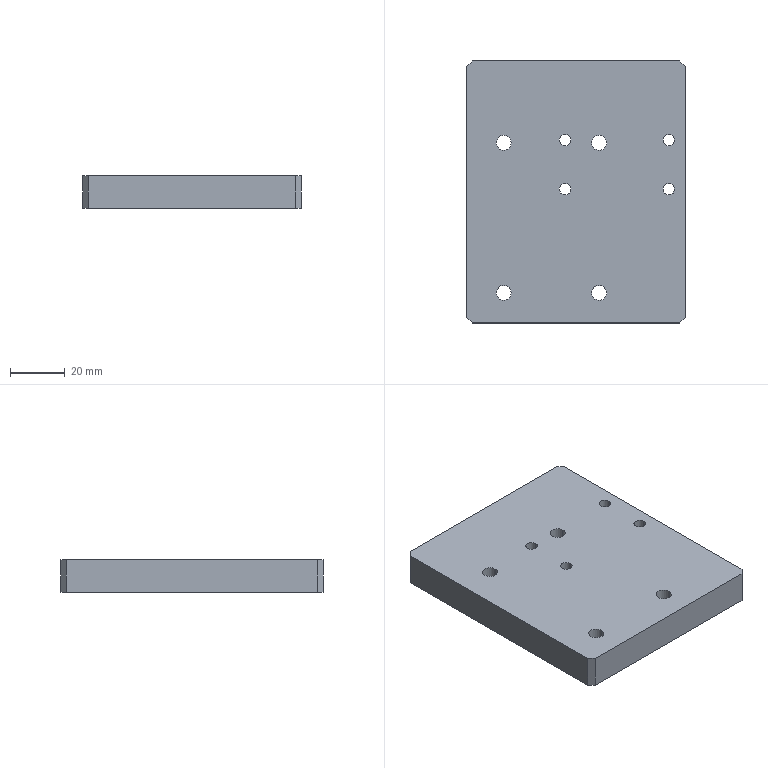CAM job | Mastercam | mm | 11 operations | part box 80 x 96 x 12
1. Facing | 20 - 63 平铣刀
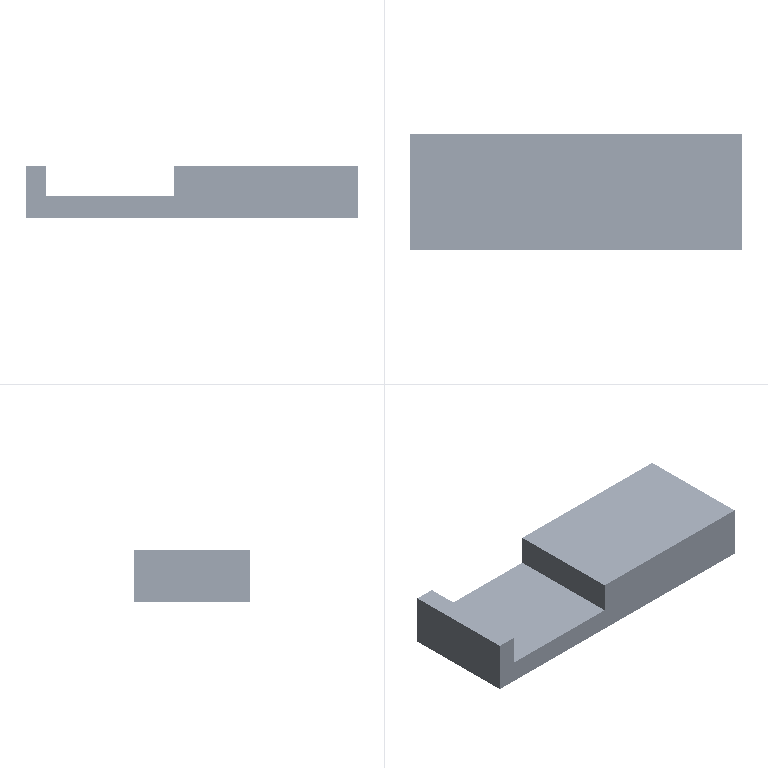2. Contour (Ramp) | 9 - 10 平铣刀
3. Contour (Ramp) | 9 - 10 平铣刀
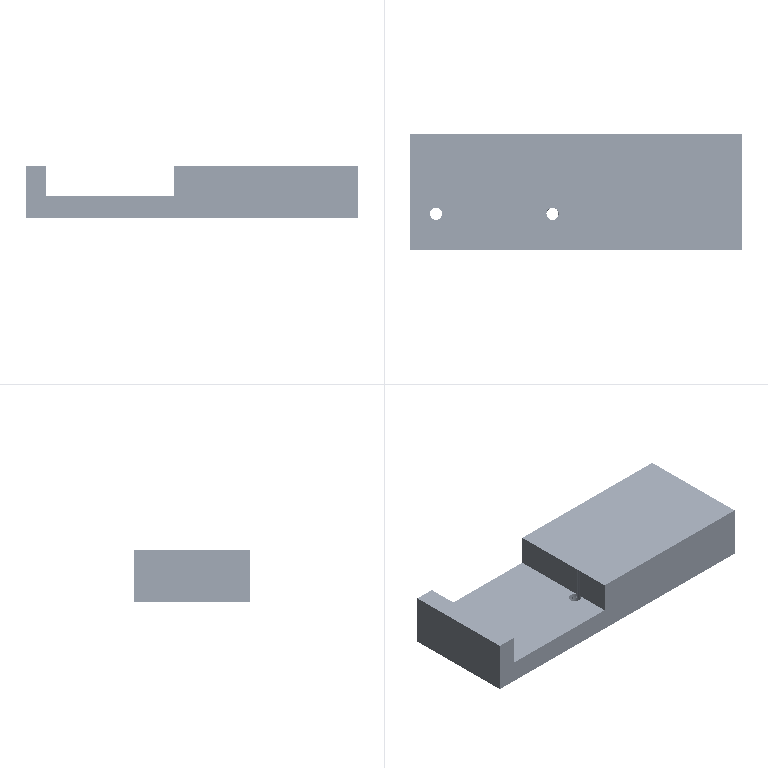4. Contour (2D) | 10 - 10 平铣刀
5. Helix Bore | 6 - 6 平铣刀
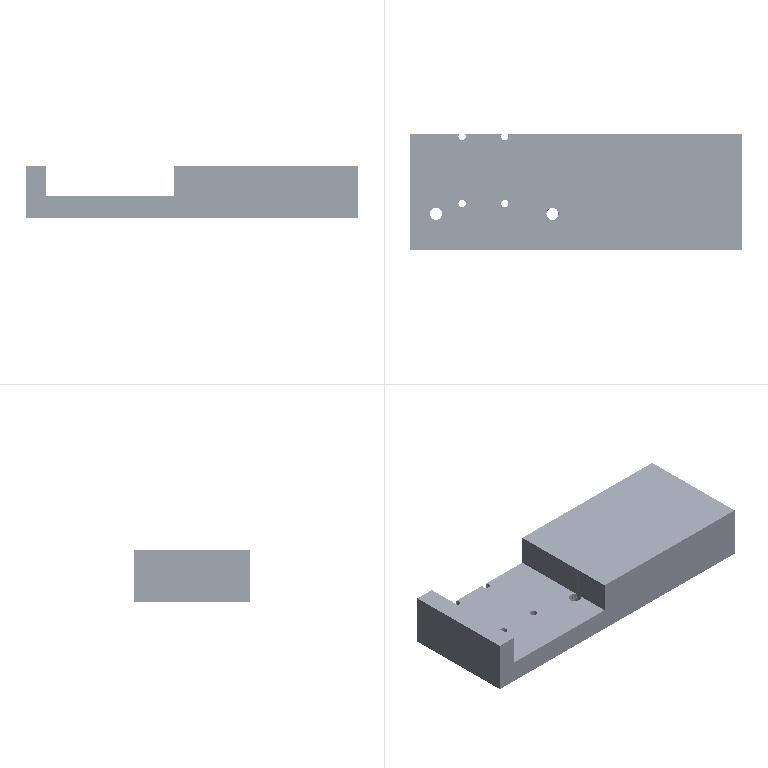6. Drill/Counterbore | 7 - 4 倒角刀
7. Contour (2D chamfer) | 7 - 4 倒角刀
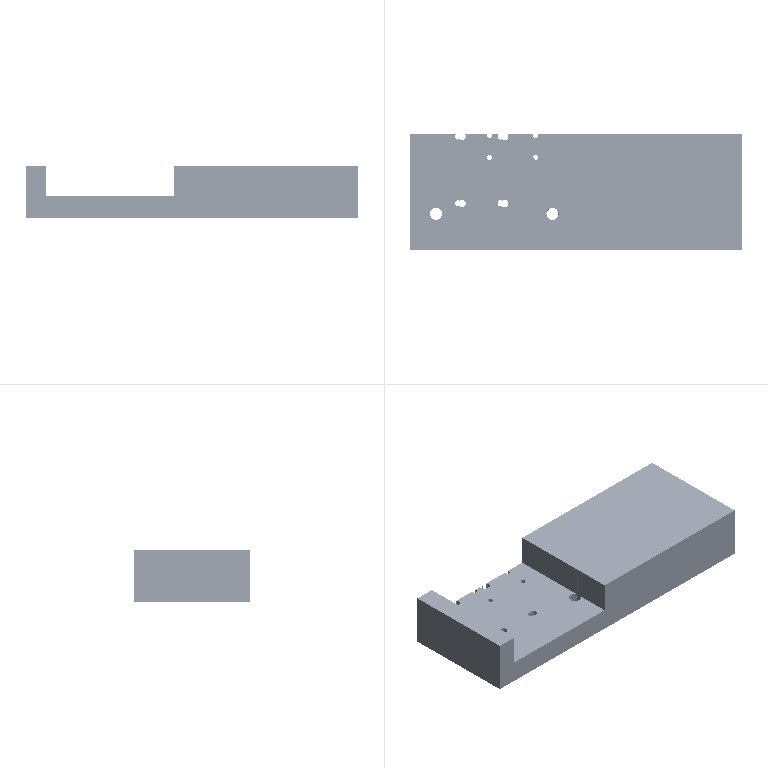8. Facing | 20 - 63 平铣刀
9. Contour (Ramp) | 9 - 10 平铣刀
10. Contour (2D) | 10 - 10 平铣刀
11. Contour (2D chamfer) | 7 - 4 倒角刀